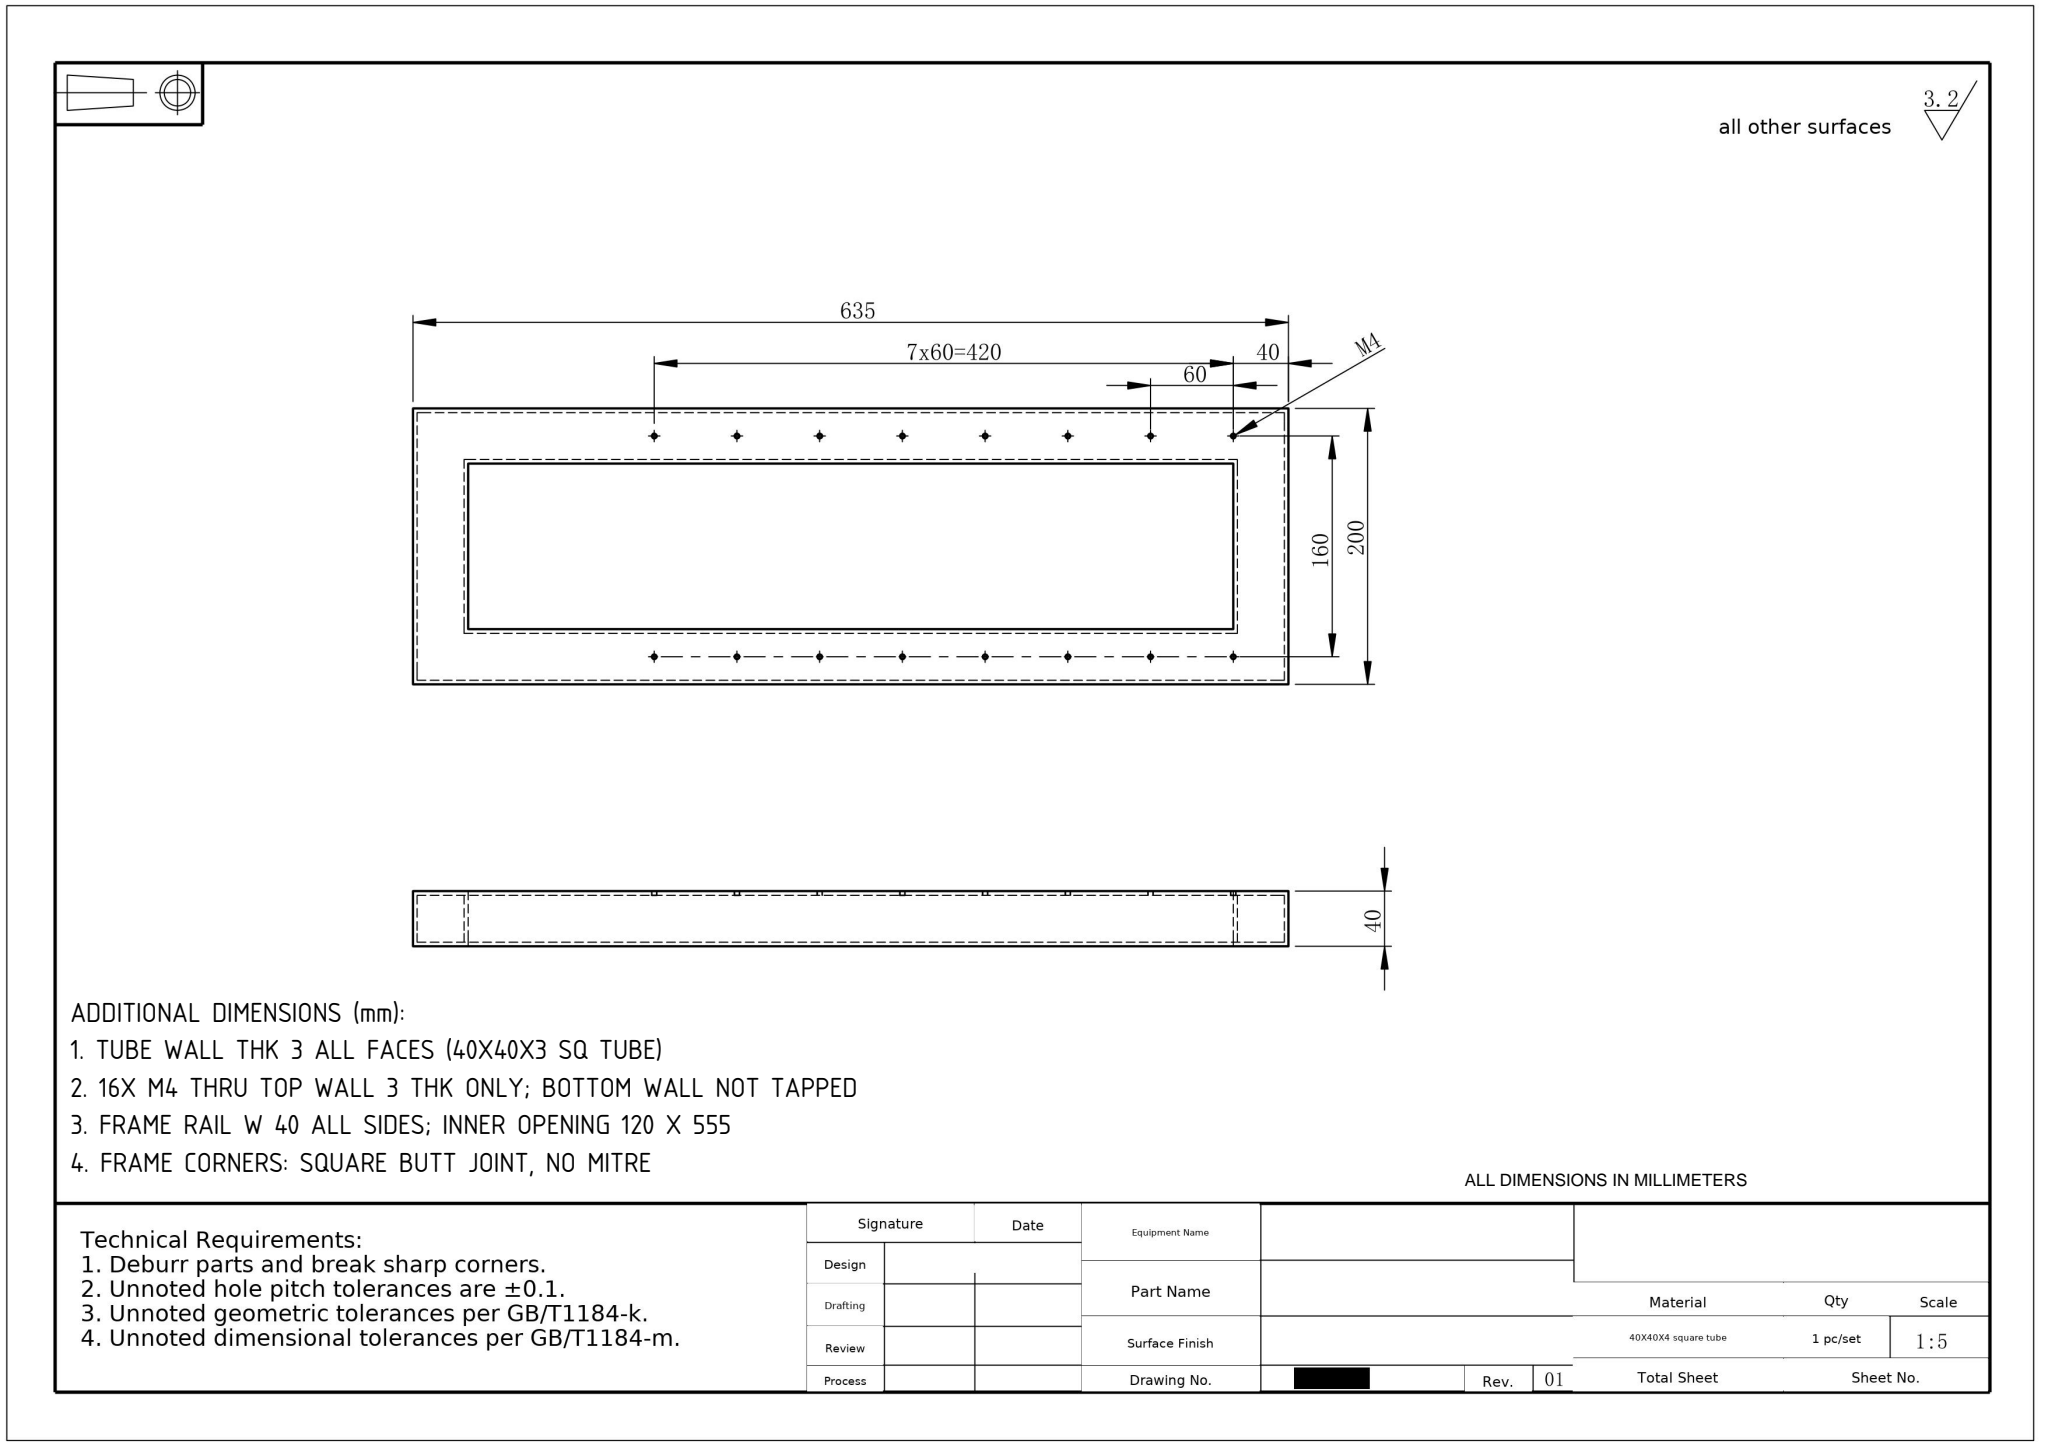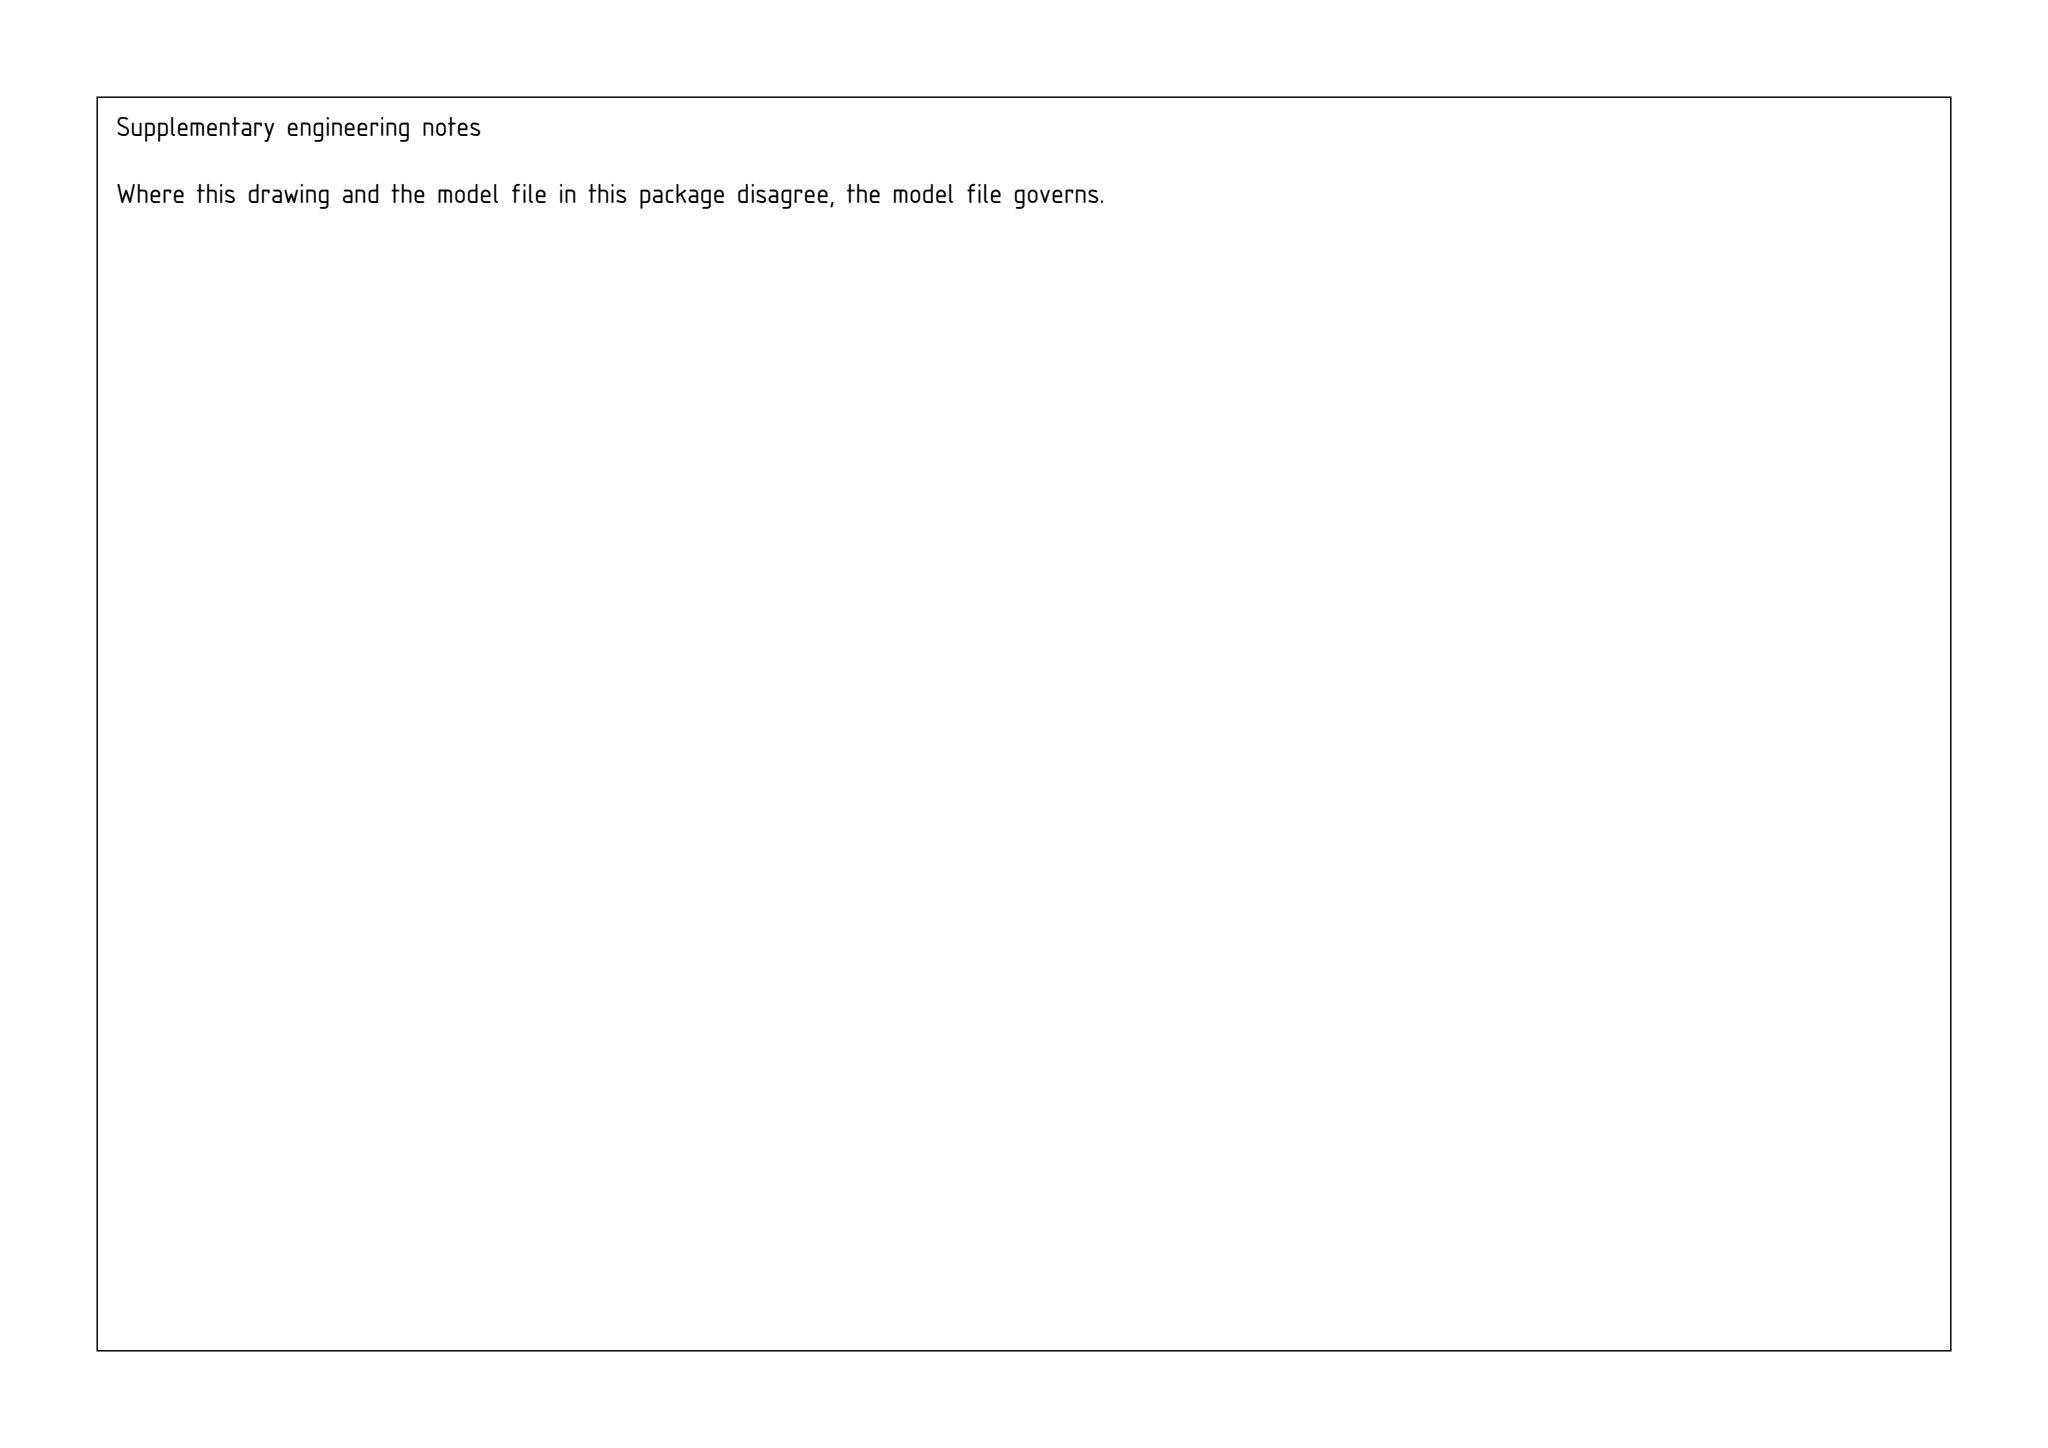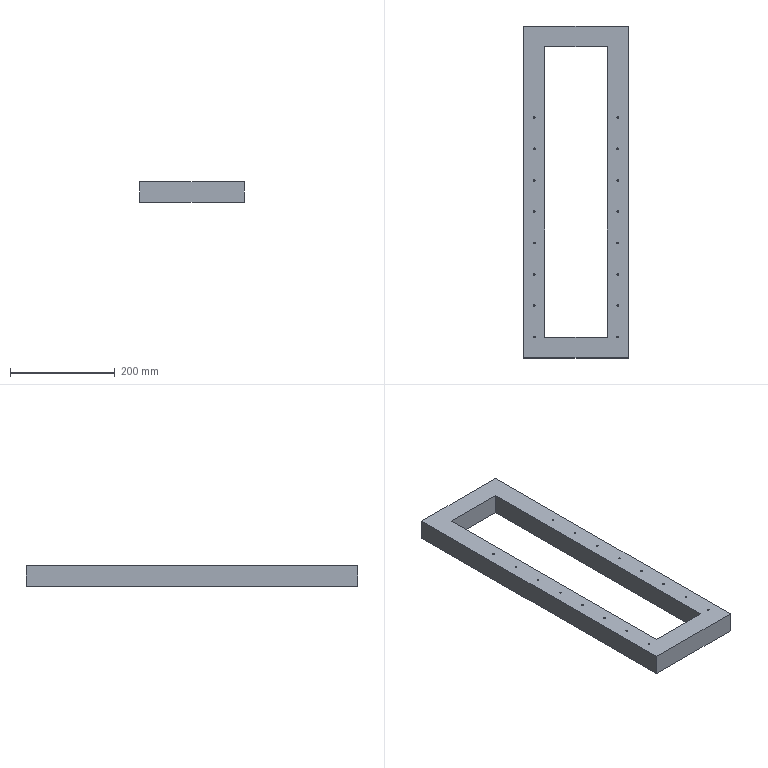Part | SolidWorks | mm | 1 solid | 52 faces | box 200 x 635 x 40 mm | volume 670029 mm3 | cylinder 32 | plane 20 | commonest cylinder face diameters 3.3 x32
build123d program:
from build123d import *

# Parameters (mm, degrees)
SKETCH1_W           = 200
SKETCH1_H           = 635
SKETCH1_W_2         = 120
SKETCH1_H_2         = 555
BOSS_EXTRUDE1_DEPTH = 40
SHELL4_T            = -3
SKETCH4_W           = 200
SKETCH4_H           = 635
SKETCH4_W_2         = 120
SKETCH4_H_2         = 555
BOSS_EXTRUDE2_DEPTH = 3
LPATTERN1_COUNT     = 8
LPATTERN1_PITCH     = 60


with BuildPart() as part:
    # Sketch1 → Boss-Extrude1 (new body)
    with BuildSketch(Plane.XY):
        Rectangle(SKETCH1_W, SKETCH1_H)
        Rectangle(SKETCH1_W_2, SKETCH1_H_2, mode=Mode.SUBTRACT)
    extrude(amount=BOSS_EXTRUDE1_DEPTH)

    # Shell4
    shell4_openings = [part.faces().sort_by_distance(p)[0] for p in [
        (0, 310.842, 0),
    ]]
    offset(amount=SHELL4_T, openings=shell4_openings, kind=Kind.INTERSECTION)

    # Sketch4 → Boss-Extrude2 (add)
    with BuildSketch(Plane(origin=(0, 0, 0), x_dir=(-1, 0, 0), z_dir=(0, 0, -1))):
        Rectangle(SKETCH4_W, SKETCH4_H)
        Rectangle(SKETCH4_W_2, SKETCH4_H_2, mode=Mode.SUBTRACT)
    extrude(amount=-BOSS_EXTRUDE2_DEPTH)

    # Sketch2 → M4 Tapped Hole1 (revolve, cut)
    with BuildSketch(Plane(origin=(-80, -277.5, 40), x_dir=(0, -1, 0), z_dir=(1, 0, 0))):
        Polygon((0, 0), (0, 12.491), (1.65, 11.5), (1.65, 0), align=None)
    m4_tapped_hole1 = revolve(axis=Axis((-80, -277.5, 46.35), (0, 0, -1)), mode=Mode.SUBTRACT)

    # LPattern1: M4 Tapped Hole1 ×8
    with Locations(*[(0, i * LPATTERN1_PITCH, 0) for i in range(1, LPATTERN1_COUNT)]):
        add(m4_tapped_hole1, mode=Mode.SUBTRACT)

    # Mirror1: M4 Tapped Hole1 across plane
    add(m4_tapped_hole1.mirror(Plane(origin=(0, 0, 0), x_dir=(0, 0, 1), z_dir=(1, 0, 0))), mode=Mode.SUBTRACT)

    # Mirror1 copy 1 sketch → Mirror1 copy 1 (revolve, cut)
    with BuildSketch(Plane(origin=(80, -217.5, 40), x_dir=(0, -1, 0), z_dir=(-1, 0, 0))):
        Polygon((0, 0), (0, -12.491), (1.65, -11.5), (1.65, 0), align=None)
    revolve(axis=Axis((80, -217.5, 46.35), (0, 0, 1)), mode=Mode.SUBTRACT)

    # Mirror1 copy 2 sketch → Mirror1 copy 2 (revolve, cut)
    with BuildSketch(Plane(origin=(80, -157.5, 40), x_dir=(0, -1, 0), z_dir=(-1, 0, 0))):
        Polygon((0, 0), (0, -12.491), (1.65, -11.5), (1.65, 0), align=None)
    revolve(axis=Axis((80, -157.5, 46.35), (0, 0, 1)), mode=Mode.SUBTRACT)

    # Mirror1 copy 3 sketch → Mirror1 copy 3 (revolve, cut)
    with BuildSketch(Plane(origin=(80, -97.5, 40), x_dir=(0, -1, 0), z_dir=(-1, 0, 0))):
        Polygon((0, 0), (0, -12.491), (1.65, -11.5), (1.65, 0), align=None)
    revolve(axis=Axis((80, -97.5, 46.35), (0, 0, 1)), mode=Mode.SUBTRACT)

    # Mirror1 copy 4 sketch → Mirror1 copy 4 (revolve, cut)
    with BuildSketch(Plane(origin=(80, -37.5, 40), x_dir=(0, -1, 0), z_dir=(-1, 0, 0))):
        Polygon((0, 0), (0, -12.491), (1.65, -11.5), (1.65, 0), align=None)
    revolve(axis=Axis((80, -37.5, 46.35), (0, 0, 1)), mode=Mode.SUBTRACT)

    # Mirror1 copy 5 sketch → Mirror1 copy 5 (revolve, cut)
    with BuildSketch(Plane(origin=(80, 22.5, 40), x_dir=(0, -1, 0), z_dir=(-1, 0, 0))):
        Polygon((0, 0), (0, -12.491), (1.65, -11.5), (1.65, 0), align=None)
    revolve(axis=Axis((80, 22.5, 46.35), (0, 0, 1)), mode=Mode.SUBTRACT)

    # Mirror1 copy 6 sketch → Mirror1 copy 6 (revolve, cut)
    with BuildSketch(Plane(origin=(80, 82.5, 40), x_dir=(0, -1, 0), z_dir=(-1, 0, 0))):
        Polygon((0, 0), (0, -12.491), (1.65, -11.5), (1.65, 0), align=None)
    revolve(axis=Axis((80, 82.5, 46.35), (0, 0, 1)), mode=Mode.SUBTRACT)

    # Mirror1 copy 7 sketch → Mirror1 copy 7 (revolve, cut)
    with BuildSketch(Plane(origin=(80, 142.5, 40), x_dir=(0, -1, 0), z_dir=(-1, 0, 0))):
        Polygon((0, 0), (0, -12.491), (1.65, -11.5), (1.65, 0), align=None)
    revolve(axis=Axis((80, 142.5, 46.35), (0, 0, 1)), mode=Mode.SUBTRACT)


solid = part.part